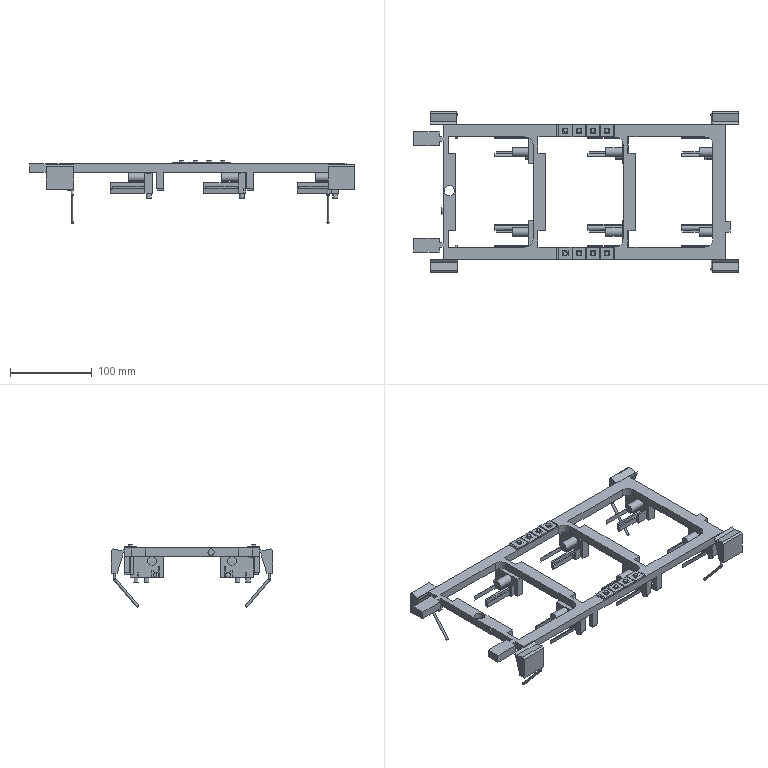Component | NX | FRAME | 19 solids | 504 faces | volume 321951 mm3 | plane 442 | cylinder 58 | torus 4 | commonest cylinder face diameters 3 x8 5 x8 6.264 x6 5.914 x6 5.65 x6 10.632 x6 20 x6 16 x6